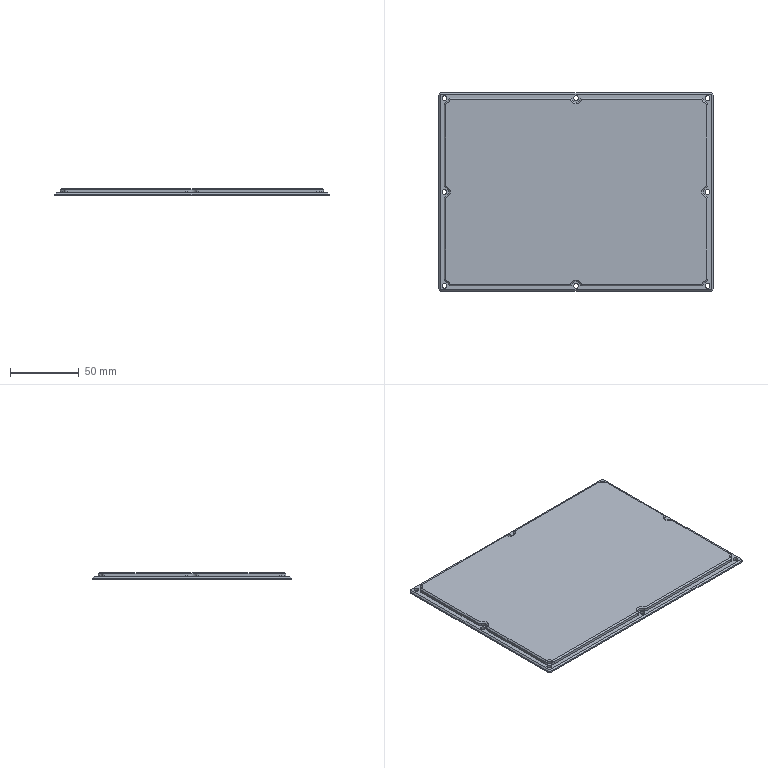CAM job | Mastercam | mm | 10 operations | part box 200 x 145 x 5
1. Contour (Ramp) | 10 - 10 平铣刀
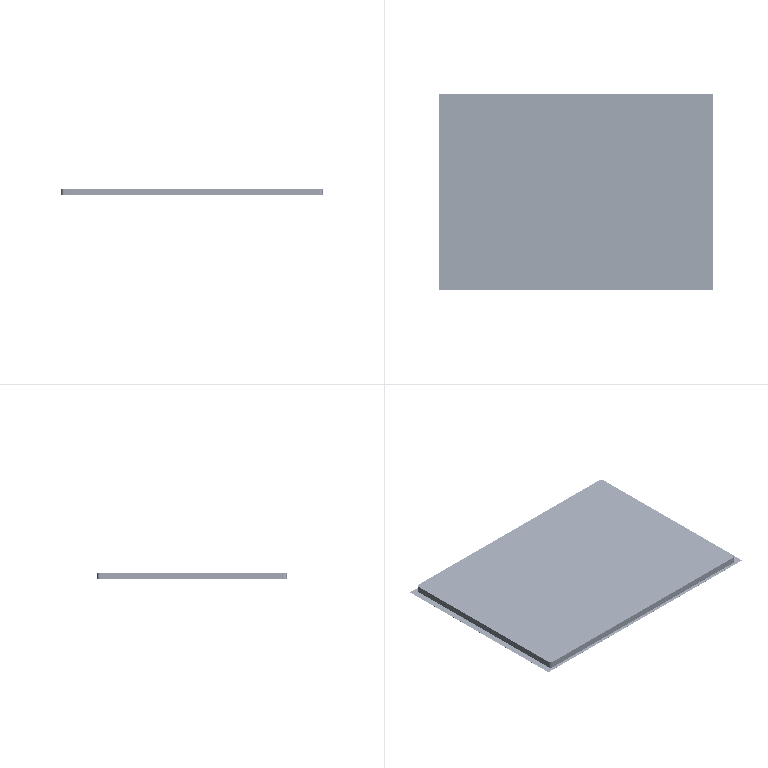2. Contour (2D) | 10 - 10 平铣刀
3. Contour (Ramp) | 6 - 6 平铣刀
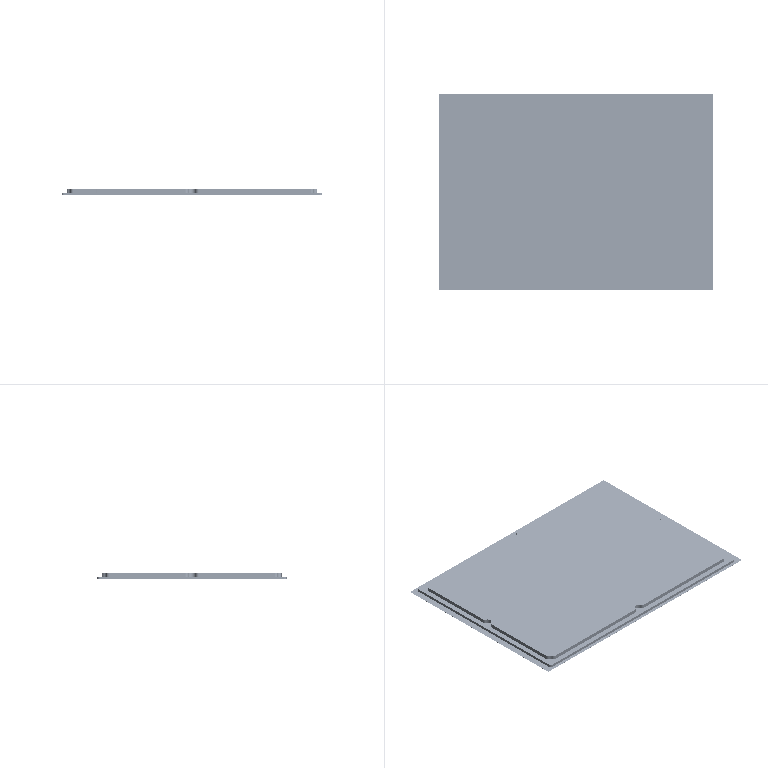4. Contour (2D) | 6 - 6 平铣刀
5. Drill/Counterbore | 7 - 4 倒角刀
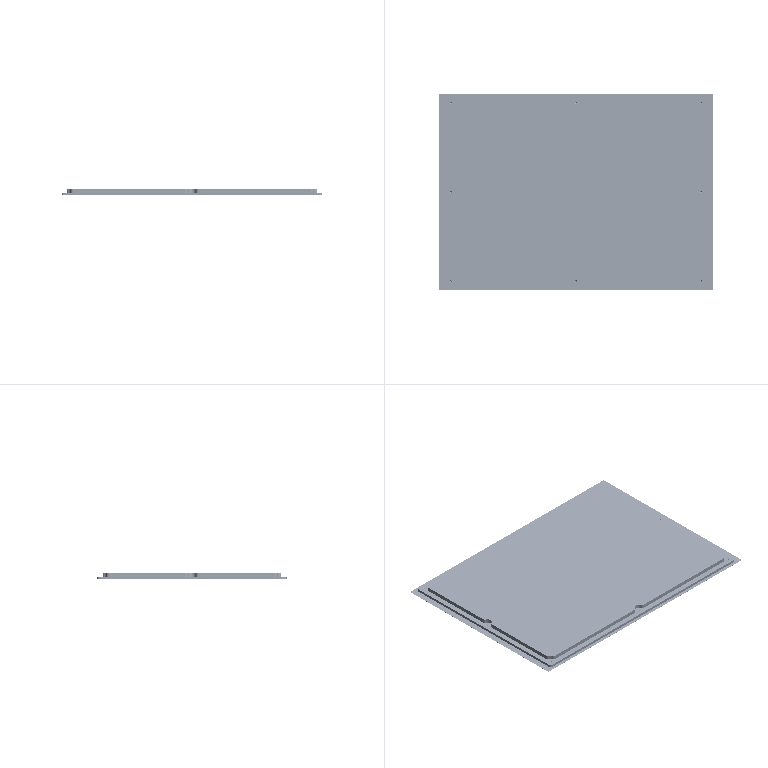6. Contour (2D chamfer) | 7 - 4 倒角刀
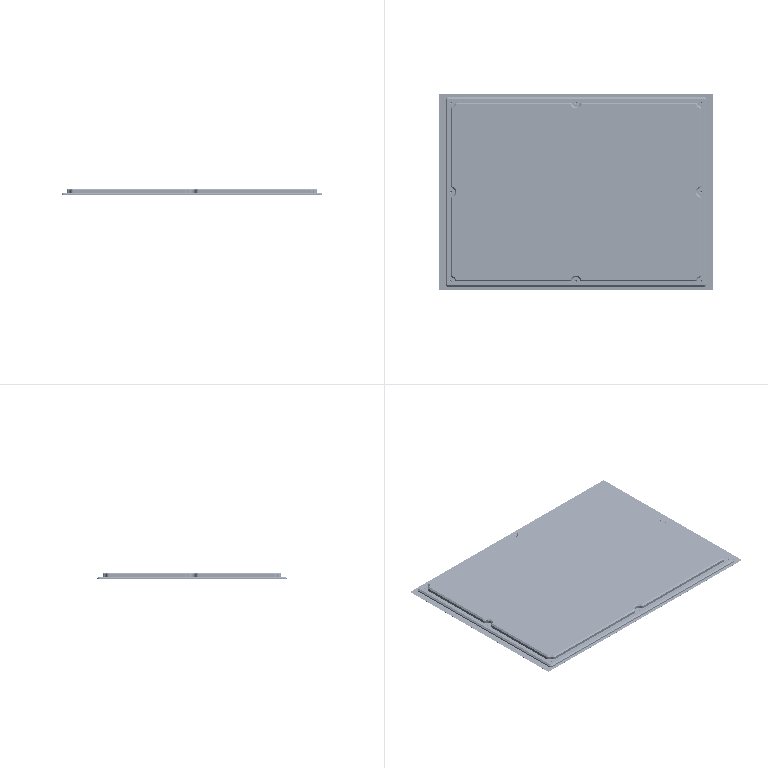7. 2D High Speed (2D Area Mill) | 6 - 6 平铣刀
8. Contour (Remachining) | 4 - 4 平铣刀
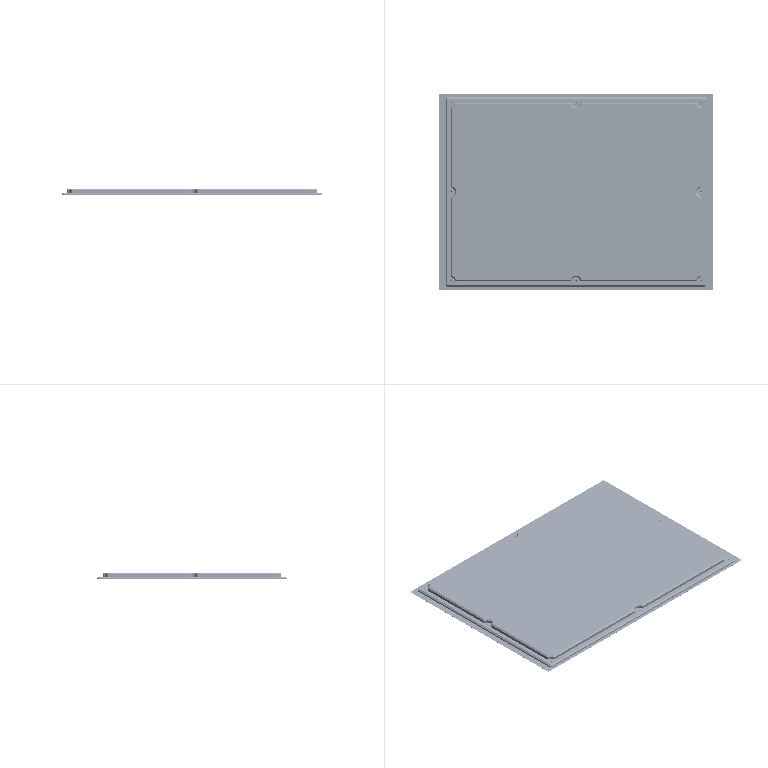9. Contour (2D) | 4 - 4 平铣刀
10. Contour (2D chamfer) | 7 - 4 倒角刀